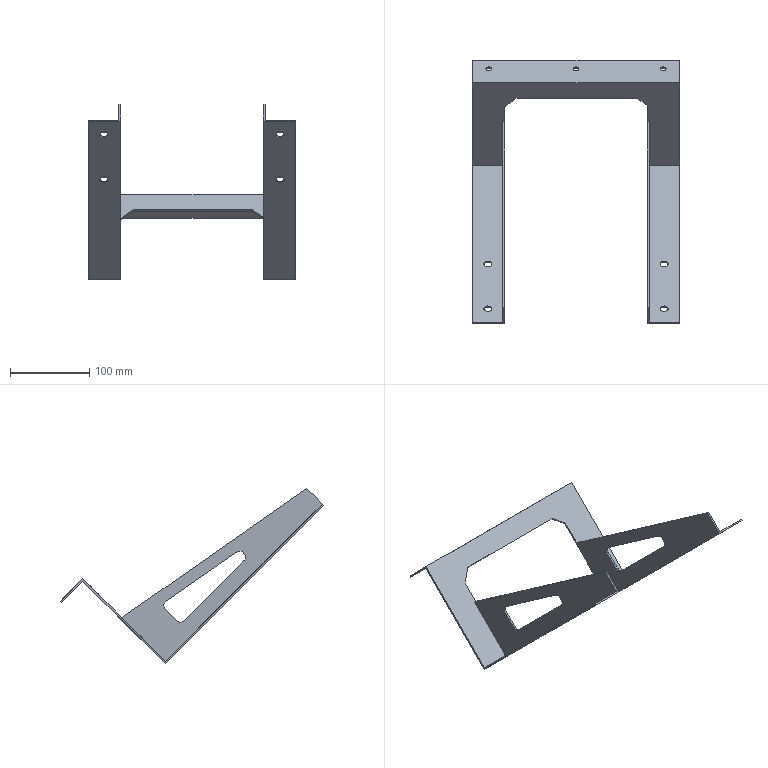Component | SolidWorks | UpperCoverBracket2-1 | 1 solid | 52 faces | box 260 x 331.63 x 220.62 mm | volume 145331 mm3 | plane 30 | cylinder 22 | commonest cylinder face diameters 10 x8 14 x8 7 x6
build123d program:
from build123d import *

# Parameters (mm, degrees)
EXTRUDE_THIN1_DEPTH = 260
SKETCH2_W           = 180
SKETCH2_H           = 282
CUT_EXTRUDE1_DEPTH  = 80
CUT_EXTRUDE2_DEPTH  = 2
BOSS_EXTRUDE1_DEPTH = 2
BOSS_EXTRUDE2_DEPTH = 2
CUT_EXTRUDE3_REACH  = 367.781
FILLET1_R           = 7
SKETCH8_R           = 5
CUT_EXTRUDE4_DEPTH  = 2
SKETCH9_R           = 3.5
CUT_EXTRUDE5_DEPTH  = 10


with BuildPart() as part:
    # Sketch1 → Extrude-Thin1 (new body)
    with BuildSketch(Plane.XY):
        Polygon((-96.672, 45.835), (-96.672, 5.835), (50.328, 5.835), (50.328, -274.165), (52.328, -274.165), (52.328, 7.835), (-94.672, 7.835), (-94.672, 45.835), align=None)
    extrude(amount=-EXTRUDE_THIN1_DEPTH)

    # Sketch2 → Cut-Extrude1 (cut)
    with BuildSketch(Plane(origin=(52.328, 0, 0), x_dir=(0, 0, -1), z_dir=(1, 0, 0))):
        with Locations((130, -133.165)):
            Rectangle(SKETCH2_W, SKETCH2_H)
    extrude(amount=-CUT_EXTRUDE1_DEPTH, mode=Mode.SUBTRACT)

    # Sketch3 → Cut-Extrude2 (cut)
    with BuildSketch(Plane(origin=(0, 7.835, 0), x_dir=(1, 0, 0), z_dir=(0, 1, 0))):
        Polygon((-27.672, 40), (-56.175, 40), (-69.672, 53.497), (-69.672, 204.329), (-54.001, 220), (-27.672, 220), align=None)
    extrude(amount=-CUT_EXTRUDE2_DEPTH, mode=Mode.SUBTRACT)

    # Sketch5 → Boss-Extrude1 (add)
    with BuildSketch(Plane(origin=(0, 0, -40), x_dir=(-1, 0, 0), z_dir=(0, 0, -1))):
        Polygon((27.672, 7.835), (-22.328, -274.165), (-52.328, -274.165), (-52.328, 7.835), align=None)
    extrude(amount=-BOSS_EXTRUDE1_DEPTH)

    # Sketch6 → Boss-Extrude2 (add)
    with BuildSketch(Plane.XY.offset(-220)):
        Polygon((52.328, -274.165), (22.328, -274.165), (-27.672, 7.835), (52.328, 7.835), align=None)
    extrude(amount=-BOSS_EXTRUDE2_DEPTH)

    # Cut-Extrude3: up to this face of the body (flat: up to its plane)
    cut_extrude3_end = Plane(part.part.faces().sort_by_distance((21.973, -112.235, -38))[0])
    # Sketch7 → Cut-Extrude3 (cut, up to the picked face)
    with BuildSketch(Plane(origin=(0, 0, -222), x_dir=(-1, 0, 0), z_dir=(0, 0, -1)), mode=Mode.PRIVATE) as cut_extrude3_sk1:
        Polygon((-30.844, -40.429), (4.156, -40.429), (-17.121, -160.429), (-30.844, -160.429), align=None)
    cut_extrude3_tool1 = split(extrude(cut_extrude3_sk1.sketch, amount=-CUT_EXTRUDE3_REACH, mode=Mode.PRIVATE), bisect_by=cut_extrude3_end, keep=Keep.BOTH, mode=Mode.PRIVATE)
    add(cut_extrude3_tool1.solids().sort_by(Axis((17.889, -91.696, -222), (0, 0, 1)))[0], mode=Mode.SUBTRACT)

    # Fillet1
    fillet1_edges = [part.edges().sort_by_distance(p)[0] for p in [
        (30.844, -160.429, -39),
        (30.844, -160.429, -221),
        (30.844, -40.429, -39),
        (30.844, -40.429, -221),
        (-4.156, -40.429, -39),
        (-4.156, -40.429, -221),
        (17.121, -160.429, -39),
        (17.121, -160.429, -221),
    ]]
    fillet(fillet1_edges, radius=FILLET1_R)

    # Sketch8 → Cut-Extrude4 (cut)
    with BuildSketch(Plane(origin=(52.328, 0, 0), x_dir=(0, 0, -1), z_dir=(1, 0, 0))):
        with Locations(Location((19, -169.868, 0), (0, 0, 90))):
            Circle(SKETCH8_R)
        with Locations(Location((19, -249.868, 0), (0, 0, 90))):
            Circle(SKETCH8_R)
        with Locations(Location((241, -249.868, 0), (0, 0, 90))):
            Circle(SKETCH8_R)
        with Locations(Location((241, -169.868, 0), (0, 0, 90))):
            Circle(SKETCH8_R)
    extrude(amount=-CUT_EXTRUDE4_DEPTH, mode=Mode.SUBTRACT)

    # Sketch9 → Cut-Extrude5 (cut)
    with BuildSketch(Plane(origin=(-94.672, 0, 0), x_dir=(0, 0, -1), z_dir=(1, 0, 0))):
        with Locations((20, 30.835)):
            Circle(SKETCH9_R)
        with Locations((130, 30.835)):
            Circle(SKETCH9_R)
        with Locations((240, 30.835)):
            Circle(SKETCH9_R)
    extrude(amount=-CUT_EXTRUDE5_DEPTH, mode=Mode.SUBTRACT)


solid = part.part

# Placed as in the assembly
solid = solid.moved(Location((248.825, 362.351, -588.779), (-45, 90, 0)))